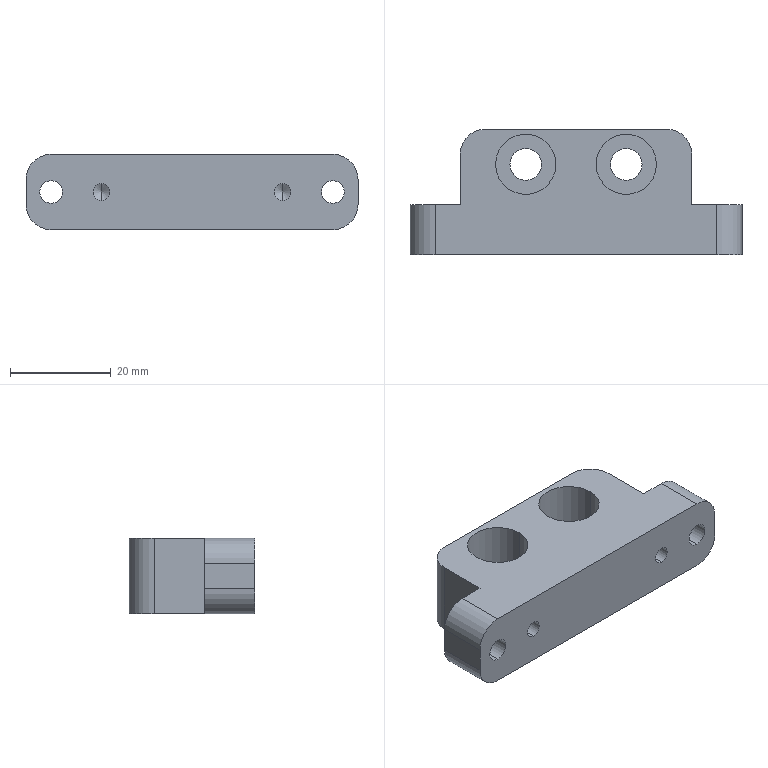Component | SolidWorks | WZH-20190520-F210StopBlockSeat-1 | 1 solid | 44 faces | box 66 x 25 x 15 mm | volume 15928 mm3 | cylinder 26 | plane 14 | cone 4 | commonest cylinder face diameters 10 x6 8 x4 4.5 x4 3.3 x4 12 x4 6.3 x4 | material 45
build123d program:
from build123d import *

# Parameters (mm, degrees)
SKETCH1_W                                         = 46
SKETCH1_H                                         = 25
BOSS_EXTRUDE1_DEPTH                               = 7.5
SKETCH2_R                                         = 3.15
CUT_EXTRUDE1_DEPTH                                = 31.17
SKETCH3_R                                         = 6
CUT_EXTRUDE2_DEPTH                                = 13
M4_TAPPED_HOLE1_D                                 = 3.3
M4_TAPPED_HOLE1_DEPTH                             = 14.1
M4_TAPPED_HOLE1_TIP                               = 0.9914
FILLET1_R                                         = 5
SKETCH6_W                                         = 10
SKETCH6_H                                         = 10
BOSS_EXTRUDE2_DEPTH                               = 15
HOLE_SIZE_ACCORDING_TO_SOCKET_HEAD_CA_D           = 4.5
HOLE_SIZE_ACCORDING_TO_SOCKET_HEAD_CA_CBORE_D     = 8
HOLE_SIZE_ACCORDING_TO_SOCKET_HEAD_CA_CBORE_DEPTH = 4.6
FILLET2_R                                         = 5


with BuildPart() as part:
    # Sketch1 → Boss-Extrude1 (new, symmetric)
    with BuildSketch(Plane.XY):
        Rectangle(SKETCH1_W, SKETCH1_H)
    extrude(amount=BOSS_EXTRUDE1_DEPTH, both=True)

    # Sketch2 → Cut-Extrude1 (cut, through all)
    with BuildSketch(Plane(origin=(0, 0, -7.5), x_dir=(-1, 0, 0), z_dir=(0, 0, -1))):
        with Locations((-10, 5.5)):
            Circle(SKETCH2_R)
        with Locations((10, 5.5)):
            Circle(SKETCH2_R)
    extrude(amount=-CUT_EXTRUDE1_DEPTH, mode=Mode.SUBTRACT)

    # Sketch3 → Cut-Extrude2 (cut)
    with BuildSketch(Plane.XY.offset(7.5)):
        with Locations((10, 5.5)):
            Circle(SKETCH3_R)
        with Locations((-10, 5.5)):
            Circle(SKETCH3_R)
    extrude(amount=-CUT_EXTRUDE2_DEPTH, mode=Mode.SUBTRACT)

    # M4 Tapped Hole1
    with Locations(Plane(origin=(0, -12.5, 0), x_dir=(-1, 0, 0), z_dir=(0, -1, 0))):
        with Locations((18, 0), (-18, 0)):
            Hole(M4_TAPPED_HOLE1_D / 2, depth=M4_TAPPED_HOLE1_DEPTH)
            with Locations((0, 0, -(M4_TAPPED_HOLE1_DEPTH + M4_TAPPED_HOLE1_TIP / 2))):  # 118° drill point
                Cone(0, M4_TAPPED_HOLE1_D / 2, M4_TAPPED_HOLE1_TIP, mode=Mode.SUBTRACT)

    # Fillet1
    fillet1_edges = [part.edges().sort_by_distance(p)[0] for p in [
        (-23, 12.5, 0),
        (23, 12.5, 0),
    ]]
    fillet(fillet1_edges, radius=FILLET1_R)

    # Sketch6 → Boss-Extrude2 (add)
    with BuildSketch(Plane.XY.offset(7.5)):
        with Locations((-28, -7.5)):
            Rectangle(SKETCH6_W, SKETCH6_H)
        with Locations((28, -7.5)):
            Rectangle(SKETCH6_W, SKETCH6_H)
    extrude(amount=-BOSS_EXTRUDE2_DEPTH)

    # Hole Size _ according to_ Socket Head Ca (through all)
    with Locations(Plane(origin=(0, -2.5, 0), x_dir=(1, 0, 0), z_dir=(0, 1, 0))):
        with Locations((-28, 0), (28, 0)):
            CounterBoreHole(HOLE_SIZE_ACCORDING_TO_SOCKET_HEAD_CA_D / 2, HOLE_SIZE_ACCORDING_TO_SOCKET_HEAD_CA_CBORE_D / 2, HOLE_SIZE_ACCORDING_TO_SOCKET_HEAD_CA_CBORE_DEPTH)

    # Fillet2
    fillet2_edges = [part.edges().sort_by_distance(p)[0] for p in [
        (-33, -7.5, 7.5),
        (-33, -7.5, -7.5),
        (33, -7.5, 7.5),
        (33, -7.5, -7.5),
    ]]
    fillet(fillet2_edges, radius=FILLET2_R)


solid = part.part